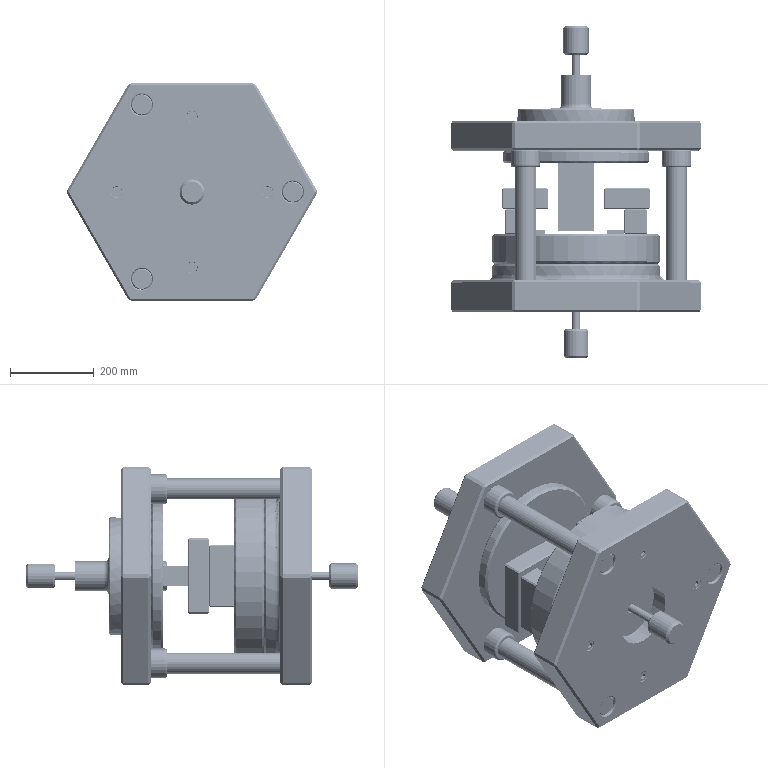Assembly | NX | mm | 43 component files | 43 solids | 1273 faces | box 595 x 792 x 519.62 mm | volume 57131856 mm3 | cylinder 574 | plane 517 | cone 100 | spline 43 | torus 39 | commonest cylinder face diameters 14 x388 10 x52 14.2 x16 25.9 x16 25.2 x16 12 x16 6 x12 18.5 x8
Bill of materials:
unnamed part 1 | 1 |  | Headed pin: a short cylindrical head with chamfered edges on one end of a long, thin, plain cylindrical shaft.
unnamed part 2 | 1 |  | Thin circular disc with chamfered rim and a rectangular block boss standing out from the centre of one face; a small hole passes through the disc centre and a small cross hole runs through the boss end.
unnamed part 3 | 2 |  | Rectangular block with chamfered edges and two pairs of closely spaced round through holes, one pair near each end of one face.
unnamed part 4 | 1 |  | Hexagonal plate with chamfered edges and a raised circular boss on one face; it has three large holes at alternate corners, four small counterbored or countersunk holes, and a small central hole.
unnamed part 5 | 1 |  | Headed pin: a cylindrical head with chamfered edges joined to a thinner plain cylindrical shaft, proportionally shorter and stockier than a long needle-like pin.
unnamed part 6 | 4 |  | Cap-head screw-like part: a cylindrical head with a round recess in its top, a plain unthreaded shank section, and a long modelled helical-thread section to the tip.
unnamed part 7 | 1 |  | Flat hexagonal plate with chamfered edges, three large holes at alternate corners, four small holes in a square pattern, and a slightly larger central hole.
unnamed part 8 | 3 |  | Plain solid cylindrical rod with small chamfers or edge breaks at both ends.
unnamed part 9 | 1 |  | Thick circular disc with chamfered edges, a central through hole, four counterbored or countersunk holes in a rectangular pattern, and four small holes near the rim at 90-degree spacing.
unnamed part 10 | 4 |  | Countersunk-head pin or rivet-like part: a conical countersunk head on a plain cylindrical shank ending in a conical point.
unnamed part 11 | 4 |  | Cap-head screw-like part: a cylindrical head with a round top recess, a long plain shank, and a short modelled thread section at the tip.
unnamed part 12 | 3 |  | Stepped tubular sleeve: a hollow cylinder with a large through bore, a larger outer diameter on one end section, and rounded or chamfered edges.
unnamed part 13 | 4 |  | Socket-head cap-screw-like part: a cylindrical head with a hexagonal recess, a plain unthreaded shank section, and a threaded section running to the tip.
unnamed part 14 | 1 |  | Flanged hub: a thin circular flange with a cylindrical boss on one side, a central through bore, and four small holes evenly spaced on a bolt circle near the rim.
unnamed part 15 | 4 |  | Long socket-head cap-screw-like part: a cylindrical head with a hexagonal recess, a long plain shank, and a shorter threaded section at the tip.
unnamed part 16 | 4 |  | Short headed threaded part: a large cylindrical head, a plain cylindrical neck, and a threaded section ending in a chamfered tip.
unnamed part 17 | 2 |  | Flat rectangular plate with a large circular-arc cutout along one edge and two through holes along the opposite edge.
unnamed part 18 | 2 |  | Rectangular block with chamfered edges and two round through holes offset toward one side of its largest face.
Mates:
1. fix | BOTTOM_PLATE 1 component
2. touch align | DIE_PLATE 1 face | BOTTOM_PLATE 1 face
3. parallel | DIE_PLATE 1 datumplane | BOTTOM_PLATE 1 face
4. touch align | BOTTOM_PLATE 1 face | DIE_PLATE 1 face
5. touch align | SUPPORTING_PLATE 2 face | DIE_PLATE 1 face
6. parallel | SUPPORTING_PLATE 2 face | BOTTOM_PLATE 1 face
7. touch align | DIE_PLATE 1 face | SUPPORTING_PLATE 2 face
8. touch align | SUPPORTING_PLATE 1 face | DIE_PLATE 1 face
9. parallel | SUPPORTING_PLATE 1 face | BOTTOM_PLATE 1 face
10. touch align | DIE_PLATE 1 face | SUPPORTING_PLATE 1 face
11. touch align | GUIDEING_PLATE 2 face | DIE_PLATE 1 face
12. parallel | GUIDEING_PLATE 2 face | BOTTOM_PLATE 1 face
13. touch align | DIE_PLATE 1 face | GUIDEING_PLATE 2 face
14. touch align | SUPPORTING_PLATE_2 2 face | SUPPORTING_PLATE 2 face
15. parallel | SUPPORTING_PLATE_2 2 face | BOTTOM_PLATE 1 face
16. touch align | SUPPORTING_PLATE 2 face | SUPPORTING_PLATE_2 2 face
17. touch align | GUIDEING_PLATE 1 face | DIE_PLATE 1 face
18. parallel | GUIDEING_PLATE 1 face | BOTTOM_PLATE 1 face
19. touch align | DIE_PLATE 1 face | GUIDEING_PLATE 1 face
20. touch align | SUPPORTING_PLATE_2 1 face | SUPPORTING_PLATE 1 face
21. parallel | SUPPORTING_PLATE_2 1 face | BOTTOM_PLATE 1 face
22. touch align | SUPPORTING_PLATE 1 face | SUPPORTING_PLATE_2 1 face
23. touch align | Guide_piller 3 face | BOTTOM_PLATE 1 face
24. parallel | Guide_piller 3 datumplane | BOTTOM_PLATE 1 face
25. distance | Guide_piller 3 face | BOTTOM_PLATE 1 face
26. distance | Guide_piller 2 face | BOTTOM_PLATE 1 face
27. parallel | Guide_piller 2 datumplane | BOTTOM_PLATE 1 face
28. touch align | Guide_piller 2 face | BOTTOM_PLATE 1 face
29. distance | Guide_piller 1 face | BOTTOM_PLATE 1 face
30. parallel | Guide_piller 1 datumplane | BOTTOM_PLATE 1 face
31. touch align | Guide_piller 1 face | BOTTOM_PLATE 1 face
32. touch align | Bush 3 face | Guide_piller 3 face
33. parallel | Bush 3 datumplane | BOTTOM_PLATE 1 face
34. distance | Guide_piller 3 face | Bush 3 face
35. fix | assembly component
36. bond | Bush 3 component | assembly component
37. bond | Bush 2 component | assembly component
38. bond | Bush 1 component | assembly component
39. circular | assembly datumaxis | assembly cartesiancoordinatesystem | assembly cartesiancoordinatesystem | assembly cartesiancoordinatesystem
40. touch align | TOP_PLATE 1 face | Bush 2 face
41. parallel | TOP_PLATE 1 face | BOTTOM_PLATE 1 face
42. touch align | Bush 2 face | TOP_PLATE 1 face
43. touch align | punch 1 face | TOP_PLATE 1 face
44. parallel | punch 1 face | BOTTOM_PLATE 1 face
45. touch align | punch 1 face | TOP_PLATE 1 face
46. touch align | shunk 1 face | TOP_PLATE 1 face
47. parallel | shunk 1 datumplane | TOP_PLATE 1 face
48. touch align | TOP_PLATE 1 face | shunk 1 face
49. touch align | alline_screw_m10 4 face | shunk 1 face
50. parallel | alline_screw_m10 4 datumplane | TOP_PLATE 1 face
51. touch align | alline_screw_m10 4 face | shunk 1 face
52. parallel | alline_screw_m10 3 datumplane | TOP_PLATE 1 face
53. touch align | alline_screw_m10 3 face | shunk 1 face
54. touch align | alline_screw_m10 3 face | shunk 1 face
55. parallel | alline_screw_m10 2 datumplane | TOP_PLATE 1 face
56. touch align | alline_screw_m10 2 face | shunk 1 face
57. touch align | alline_screw_m10 2 face | shunk 1 face
58. parallel | alline_screw_m10 1 datumplane | TOP_PLATE 1 face
59. touch align | alline_screw_m10 1 face | shunk 1 face
60. touch align | alline_screw_m10 1 face | shunk 1 face
61. touch align | ejector1 1 face | shunk 1 face
62. parallel | ejector1 1 datumplane | TOP_PLATE 1 face
63. distance | ejector1 1 face | punch 1 face
64. touch align | ejector2 1 face | BOTTOM_PLATE 1 face
65. parallel | ejector2 1 datumplane | BOTTOM_PLATE 1 face
66. distance | ejector2 1 face | DIE_PLATE 1 face
67. touch align | alline_screw_m14_t_2_ph 4 face | TOP_PLATE 1 face
68. parallel | alline_screw_m14_t_2_ph 4 datumplane | TOP_PLATE 1 face
69. touch align | alline_screw_m14_t_2_ph 4 face | TOP_PLATE 1 face
70. touch align | alline_screw_m14_t_2_ph 3 face | TOP_PLATE 1 face
71. touch align | alline_screw_m14_t_2_ph 3 face | TOP_PLATE 1 face
72. parallel | alline_screw_m14_t_2_ph 3 datumplane | TOP_PLATE 1 face
73. touch align | alline_screw_m14_t_2_ph 2 face | TOP_PLATE 1 face
74. touch align | alline_screw_m14_t_2_ph 2 face | TOP_PLATE 1 face
75. parallel | alline_screw_m14_t_2_ph 2 datumplane | TOP_PLATE 1 face
76. touch align | alline_screw_m14_t_2_ph 1 face | TOP_PLATE 1 face
77. touch align | alline_screw_m14_t_2_ph 1 face | TOP_PLATE 1 face
78. parallel | alline_screw_m14_t_2_ph 1 datumplane | TOP_PLATE 1 face
79. touch align | alline_screw_m14_sup_2_sup1 4 face | SUPPORTING_PLATE_2 1 face
80. parallel | alline_screw_m14_sup_2_sup1 4 datumplane | BOTTOM_PLATE 1 face
81. touch align | alline_screw_m14_sup_2_sup1 4 face | SUPPORTING_PLATE_2 1 face
82. touch align | alline_screw_m14_sup_2_sup1 3 face | SUPPORTING_PLATE_2 1 face
83. parallel | alline_screw_m14_sup_2_sup1 3 datumplane | BOTTOM_PLATE 1 face
84. touch align | alline_screw_m14_sup_2_sup1 3 face | SUPPORTING_PLATE_2 1 face
85. touch align | alline_screw_m14_sup_2_sup1 2 face | SUPPORTING_PLATE_2 2 face
86. parallel | alline_screw_m14_sup_2_sup1 2 datumplane | BOTTOM_PLATE 1 face
87. touch align | alline_screw_m14_sup_2_sup1 2 face | SUPPORTING_PLATE_2 2 face
88. touch align | alline_screw_m14_sup_2_sup1 1 face | SUPPORTING_PLATE_2 2 face
89. parallel | alline_screw_m14_sup_2_sup1 1 datumplane | BOTTOM_PLATE 1 face
90. touch align | SUPPORTING_PLATE_2 2 face | alline_screw_m14_sup_2_sup1 1 face
91. touch align | sp_2sp1 4 face | GUIDEING_PLATE 1 face
92. parallel | sp_2sp1 4 face | GUIDEING_PLATE 1 face
93. touch align | GUIDEING_PLATE 1 face | sp_2sp1 4 face
94. touch align | GUIDEING_PLATE 1 face | sp_2sp1 3 face
95. parallel | sp_2sp1 3 face | GUIDEING_PLATE 1 face
96. touch align | sp_2sp1 3 face | GUIDEING_PLATE 1 face
97. touch align | sp_2sp1 2 face | GUIDEING_PLATE 2 face
98. parallel | sp_2sp1 2 face | GUIDEING_PLATE 2 face
99. touch align | sp_2sp1 2 face | GUIDEING_PLATE 2 face
100. touch align | sp_2sp1 1 face | GUIDEING_PLATE 2 face
101. touch align | sp_2sp1 1 face | GUIDEING_PLATE 2 face
102. parallel | sp_2sp1 1 face | GUIDEING_PLATE 2 face
103. touch align | alline_screw_m14_dp_2_sp 4 face | DIE_PLATE 1 face
104. parallel | alline_screw_m14_dp_2_sp 4 datumplane | TOP_PLATE 1 face
105. touch align | alline_screw_m14_dp_2_sp 4 face | DIE_PLATE 1 face
106. touch align | alline_screw_m14_dp_2_sp 3 face | DIE_PLATE 1 face
107. parallel | alline_screw_m14_dp_2_sp 3 datumplane | TOP_PLATE 1 face
108. touch align | alline_screw_m14_dp_2_sp 3 face | DIE_PLATE 1 face
109. touch align | alline_screw_m14_dp_2_sp 2 face | DIE_PLATE 1 face
110. parallel | alline_screw_m14_dp_2_sp 2 datumplane | TOP_PLATE 1 face
111. touch align | alline_screw_m14_dp_2_sp 2 face | DIE_PLATE 1 face
112. touch align | alline_screw_m14_dp_2_sp 1 face | DIE_PLATE 1 face
113. parallel | alline_screw_m14_dp_2_sp 1 datumplane | TOP_PLATE 1 face
114. touch align | alline_screw_m14_dp_2_sp 1 face | DIE_PLATE 1 face
115. touch align | alline_screw_m14_bp_2_dp 4 face | BOTTOM_PLATE 1 face
116. parallel | alline_screw_m14_bp_2_dp 4 datumplane | BOTTOM_PLATE 1 face
117. touch align | BOTTOM_PLATE 1 face | alline_screw_m14_bp_2_dp 4 face
118. parallel | alline_screw_m14_bp_2_dp 3 datumplane | BOTTOM_PLATE 1 face
119. touch align | BOTTOM_PLATE 1 face | alline_screw_m14_bp_2_dp 3 face
120. touch align | alline_screw_m14_bp_2_dp 3 face | BOTTOM_PLATE 1 face
121. parallel | alline_screw_m14_bp_2_dp 2 datumplane | BOTTOM_PLATE 1 face
122. touch align | BOTTOM_PLATE 1 face | alline_screw_m14_bp_2_dp 2 face
123. touch align | alline_screw_m14_bp_2_dp 2 face | BOTTOM_PLATE 1 face
124. parallel | alline_screw_m14_bp_2_dp 1 datumplane | BOTTOM_PLATE 1 face
125. touch align | BOTTOM_PLATE 1 face | alline_screw_m14_bp_2_dp 1 face
126. touch align | alline_screw_m14_bp_2_dp 1 face | BOTTOM_PLATE 1 face